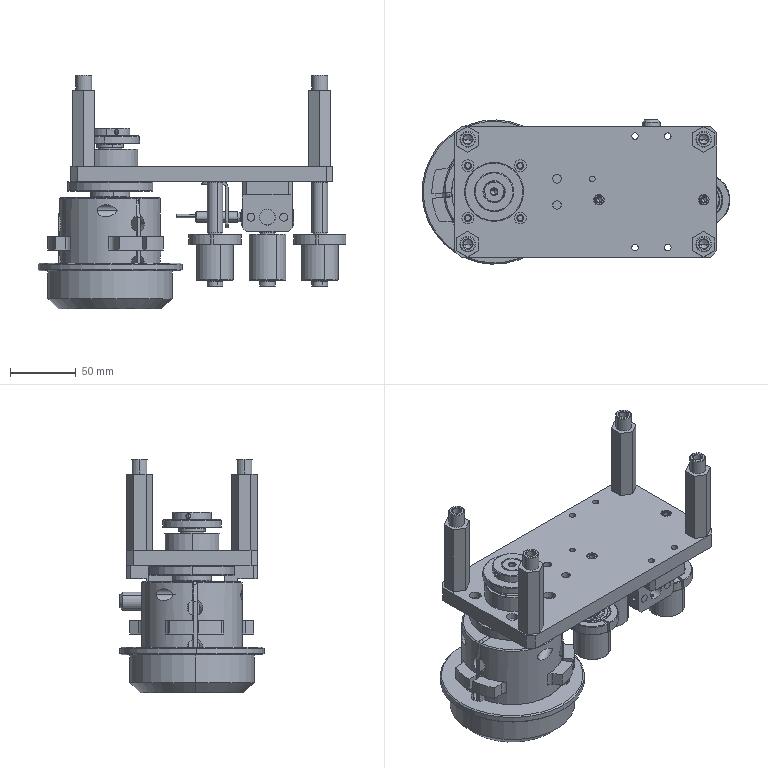Assembly | SolidWorks | mm | 39 component files | 95 solids | 1291 faces | box 235 x 110 x 178.5 mm | volume 896661 mm3 | cylinder 488 | plane 301 | cone 285 | spline 214 | torus 3 | commonest cylinder face diameters 12 x89 4.2 x28 9 x26 3.3 x26 24 x24 19.68 x24 16.32 x24 5 x22
Bill of materials:
61901Bearing | 6 | 45#Steel | Annular assembly of concentric outer and inner rings with flat faces, separated by an open annular gap holding six spherical elements spaced around it; looks like an open (unshielded) ball-bearing shape.
61904Bearing | 2 | 45#Steel | Same type of shape as the previous part: concentric inner and outer rings with six spheres in the annular gap between them, forming an open ball-bearing-like ring set.
YX-04-110GluePaperFeedingPressureRollerAxis | 2 | Hard Chrome Rod | Long stepped cylindrical shaft with a shorter, smaller-diameter end and an axial blind bore in the small end. The larger body has two narrow circumferential grooves: one around mid-length and one near the far end.
YX-04-111GluePaperRetainingRing | 2 | 45#Steel | Flat split ring with a rectangular cross-section, a single radial cut through the ring, and chamfered edges; looks like a split washer or split collar.
YX-04-112GluePaperFeedingBearingFixingSleeve | 3 | 45#Steel | Thin-walled cylindrical sleeve or bushing with an internal step near one end: a slightly larger counterbore at the top opening and a through bore.
YX-04-113GluePaperFeedingTensioningWheelFixingBlock | 2 | 45#Steel | Prismatic block with an L-shaped side profile. The top flange has two vertical through holes. The front face has one large central hole flanked by two medium holes. There are additional small holes, including one on the side leg, and chamfers on the lower corners.
YX-04-114GluePaperFeedingTensioningWheelAdjustingPost | 1 | 45#Steel | Stepped hollow cylindrical bushing or spacer: a larger-diameter body with a chamfer at one end and a smaller-diameter neck at the other. The axial bore opens at the small end.
YX-04-115GluePaperFeedingTensioningWheelGuideSleeve | 2 | Brass | Plain cylindrical tube or spacer with a concentric through bore and chamfered outer edges at both ends.
YX-04-116GluePaperFeedingTensioningWheelGuidePost | 2 | Hard Chrome Rod | Slender solid cylindrical rod or pin with plain flat ends and very small edge breaks.
YX-04-117GluePaperFeedingTensioningWheelFixingPlate | 1 | 45#Steel | Rectangular block with chamfered long edges, two large parallel through bores along one axis, and one smaller through hole on a perpendicular axis set midway between them.
YX-04-118GluePaperFeedingTensioningWheelAxis | 1 | 45#Steel | Stepped cylindrical shaft with a smaller-diameter end portion containing an axial bore, and a larger main body with narrow circumferential grooves near both ends.
PR8-2DN_1ProximitySwitch | 1 | 45#Steel | Solid stepped cylindrical rod: a thin small-diameter pin extending from a larger cylindrical body, which ends in a short, slightly reduced-diameter pilot step with a chamfer.
YX-04-102GluePaperFeedingColumn | 4 | Brass | Long hexagonal prism body with a shorter, smaller-diameter cylindrical boss coaxial at each end; a bore runs in from the top boss end, and the end view shows a recessed hole with a conical bottom.
YX-04-103GluePaperFeedingBottomPlate | 1 | 45#Steel | Flat rectangular plate with small chamfered corners, a large circular through-opening near one end, and many smaller through-holes of several sizes.
YX-04-104GluePaperFeedingBearingFixingSeat | 1 | 45#Steel | Flanged cylindrical sleeve: a thin round flange with four through-holes evenly spaced on a circle, and a taller hollow cylinder rising from it with an internal step in the bore.
YX-04-105GluePaperFeedingSensingBlock | 1 | 45#Steel | Stepped round hub: a wide thin disc with a smaller coaxial cylindrical boss on top, a central through-bore, and radial holes through the boss wall.
YX-04-106GluePaperFeedingRotatingAxis | 1 | 45#Steel | Stepped cylindrical shaft or pin with a thin integral collar near mid-length, a smaller-diameter pilot at the top end with a small axial hole, and a narrow groove or step near the upper shoulder.
YX-04-107GluePaperFeedingExpansionAxis | 1 | 45#Steel | Cylindrical body with a central axial bore, three outward-projecting lugs at mid-height, three radial slots on the top face, an axial slit through the side, a circumferential slot, and several radial and transverse holes.
YX-04-108GluePaperFeedingExpansionAxisCoverPlate | 1 | 45#Steel | Shallow round cup or cap with an outer lip flange at the top, a chamfered bottom edge, an internal cylindrical recess with two semicircular notches at its rim, and a small central hole in the floor.
YX-04-109GluePaperFeedingExpansionPlate | 3 | Delrin | Flat bar plate with two obround slots near the ends; one long edge is tapered toward each end and the corners on that side are rounded.
YX-04-119GlueFeedingProximitySwitchFixingPlate | 1 | SUS340 | L-shaped bracket bent from flat stock with a rounded inside bend; one leg has an elongated slot, the other a single round hole, and the free corners are rounded.
Mates:
1. concentric | YX-04-103GluePaperFeedingBottomPlate-1 face at (-123.397, -33.738, 194) dir (0, 0, -1) r 6 | YX-04-102GluePaperFeedingColumn-1 face at (-123.397, -33.738, 264) dir (0, 0, 1) r 6
2. concentric | YX-04-106GluePaperFeedingRotatingAxis-1 face at (-103.397, 6.262, 112) dir (0, 0, 1) r 10 | YX-04-107GluePaperFeedingExpansionAxis-1 face at (-103.397, 6.262, 182) dir (0, 0, 1) r 10
3. coincident | YX-04-106GluePaperFeedingRotatingAxis-1 face at (-103.397, 6.262, 112) dir (0, 0, -1) | YX-04-107GluePaperFeedingExpansionAxis-1 face at (-103.397, 6.262, 112) dir (0, 0, -1)
4. concentric | YX-04-106GluePaperFeedingRotatingAxis-1 face at (-103.397, 6.262, 112) dir (0, 0, -1) r 3.4 | YX-04-108GluePaperFeedingExpansionAxisCoverPlate-1 face at (-103.397, 6.262, 97) dir (0, 0, -1) r 4.5
5. width | YX-04-109GluePaperFeedingExpansionPlate-1 face at (-86.886, 36.162, 179) dir (0.8958, -0.4445, 0) | YX-04-109GluePaperFeedingExpansionPlate-1 face at (-89.573, 37.496, 179) dir (-0.8958, 0.4445, 0) | YX-04-107GluePaperFeedingExpansionAxis-1 face at (-75.16, 59.231, 112) dir (-0.8958, 0.4445, 0) | YX-04-107GluePaperFeedingExpansionAxis-1 face at (-96.075, 24.955, 112) dir (0.8958, -0.4445, 0)
6. width | YX-04-109GluePaperFeedingExpansionPlate-1 face at (-87.348, 35.23, 124.5) dir (0, 0, -1) | YX-04-109GluePaperFeedingExpansionPlate-1 face at (-88.682, 32.543, 119.5) dir (0, 0, 1) | YX-04-107GluePaperFeedingExpansionAxis-1 face at (-64.224, 20.314, 122) dir (0.8958, -0.4445, 0) r 2.75
7. coincident | YX-04-107GluePaperFeedingExpansionAxis-1 face at (-103.397, 6.262, 112) dir (0, 0, -1) | YX-04-109GluePaperFeedingExpansionPlate-1 face at (-86.886, 36.162, 112) dir (0, 0, -1)
8. coincident | YX-04-103GluePaperFeedingBottomPlate-1 face at (-33.397, 6.262, 206) dir (0, 0, 1) | YX-04-102GluePaperFeedingColumn-1 face at (-123.397, -33.738, 206) dir (0, 0, -1)
9. concentric | YX-04-106GluePaperFeedingRotatingAxis-1 face at (-103.397, 6.262, 235) dir (0, 0, -1) r 8 | YX-04-105GluePaperFeedingSensingBlock-1 face at (-103.397, 6.262, 235) dir (0, 0, 1) r 8
10. coincident | YX-04-103GluePaperFeedingBottomPlate-1 face at (-33.397, 6.262, 194) dir (0, 0, -1) | GluePaperFeedingPressureRollerAssembly-1/YX-04-110GluePaperFeedingPressureRollerAxis-1 face at (-18.121, 1.815, 194) dir (0, 0, 1)
11. concentric | YX-04-103GluePaperFeedingBottomPlate-1 face at (-23.397, 0.262, 194) dir (0, 0, -1) r 4 | GluePaperFeedingPressureRollerAssembly-1/YX-04-110GluePaperFeedingPressureRollerAxis-1 face at (-23.397, 0.262, 205.5) dir (0, 0, -1) r 6
12. coincident | YX-04-103GluePaperFeedingBottomPlate-1 face at (-33.397, 6.262, 194) dir (0, 0, -1) | GluePaperFeedingTensioningWheelAssembly-1/YX-04-113GluePaperFeedingTensioningWheelFixingBlock-2 face at (-2.397, 31.262, 194) dir (0, 0, 1)
13. concentric | YX-04-103GluePaperFeedingBottomPlate-1 face at (4.103, 48.762, 194) dir (0, 0, -1) r 2.5 | GluePaperFeedingTensioningWheelAssembly-1/YX-04-113GluePaperFeedingTensioningWheelFixingBlock-2 face at (4.103, 48.762, 194) dir (0, 0, 1) r 3.25
14. concentric | YX-04-103GluePaperFeedingBottomPlate-1 face at (29.103, 48.762, 194) dir (0, 0, -1) r 2.5 | GluePaperFeedingTensioningWheelAssembly-1/YX-04-113GluePaperFeedingTensioningWheelFixingBlock-2 face at (29.103, 48.762, 184) dir (0, 0, -1) r 3.25
15. coincident | YX-04-103GluePaperFeedingBottomPlate-1 face at (-33.397, 6.262, 194) dir (0, 0, -1) | YX-04-119GlueFeedingProximitySwitchFixingPlate-1 face at (-13.397, 14.462, 194) dir (0, 0, 1)
16. width | YX-04-119GlueFeedingProximitySwitchFixingPlate-1 face at (-25.797, 21.962, 159) dir (-1, 0, 0) | YX-04-119GlueFeedingProximitySwitchFixingPlate-1 face at (-30.997, 31.962, 159) dir (1, 0, 0) | YX-04-103GluePaperFeedingBottomPlate-1 face at (-28.397, 16.262, 194) dir (0, 0, -1) r 2.1
17. parallel | GluePaperFeedingTensioningWheelAssembly-1/YX-04-113GluePaperFeedingTensioningWheelFixingBlock-2 face at (-2.397, 31.262, 156) dir (-1, 0, 0) | YX-04-119GlueFeedingProximitySwitchFixingPlate-1 face at (-33.397, 26.962, 194) dir (-1, 0, 0)
18. distance | YX-04-103GluePaperFeedingBottomPlate-1 face at (-28.397, 16.262, 194) dir (0, 0, -1) r 2.1 | YX-04-119GlueFeedingProximitySwitchFixingPlate-1 face at (-28.397, 21.962, 159) dir (0, 0, 1) r 2.6
19. concentric | YX-04-119GlueFeedingProximitySwitchFixingPlate-1 face at (-13.397, 26.962, 167) dir (1, 0, 0) r 4.25 | PR8-2DN_1ProximitySwitch-1 face at (-5.897, 26.962, 167) dir (-1, 0, 0) r 4
20. distance | PR8-2DN_1ProximitySwitch-1 face at (-3.397, 26.962, 167) dir (1, 0, 0) | YX-04-119GlueFeedingProximitySwitchFixingPlate-1 face at (-13.397, 26.962, 194) dir (1, 0, 0)
21. coincident | GluePaperFeedingTensioningWheelAssembly-1/YX-04-112GluePaperFeedingBearingFixingSleeve-1 face at (26.976, 26.795, 125) dir (0, 0, -1) | 61901Bearing-2 face at (16.603, 20.762, 125) dir (0, 0, 1)
22. concentric | GluePaperFeedingTensioningWheelAssembly-1/YX-04-112GluePaperFeedingBearingFixingSleeve-1 face at (16.603, 20.762, 119) dir (0, 0, 1) r 12 | 61901Bearing-2 face at (16.603, 20.762, 118.7) dir (0, 0, 1) r 12
23. coincident | GluePaperFeedingTensioningWheelAssembly-1/YX-04-118GluePaperFeedingTensioningWheelAxis-1 face at (16.603, 26.762, 154) dir (0, 0, 1) | 61901Bearing-3 face at (16.603, 20.762, 154) dir (0, 0, 1)
24. concentric | GluePaperFeedingTensioningWheelAssembly-1/YX-04-118GluePaperFeedingTensioningWheelAxis-1 face at (16.603, 20.762, 174) dir (0, 0, -1) r 6 | 61901Bearing-3 face at (16.603, 20.762, 147.7) dir (0, 0, 1) r 6
25. coincident | YX-04-104GluePaperFeedingBearingFixingSeat-1 face at (-103.397, 22.262, 210) dir (0, 0, 1) | 61904Bearing-1 face at (-103.397, 6.262, 210) dir (0, 0, -1)
26. concentric | YX-04-104GluePaperFeedingBearingFixingSeat-1 face at (-103.397, 6.262, 219) dir (0, 0, -1) r 18.5 | 61904Bearing-1 face at (-103.397, 6.262, 219.45) dir (0, 0, -1) r 18.5
27. coincident | YX-04-104GluePaperFeedingBearingFixingSeat-1 face at (-103.397, 24.762, 196) dir (0, 0, -1) | 61904Bearing-2 face at (-103.397, 6.262, 196) dir (0, 0, 1)
28. concentric | YX-04-104GluePaperFeedingBearingFixingSeat-1 face at (-103.397, 6.262, 219) dir (0, 0, -1) r 18.5 | 61904Bearing-2 face at (-103.397, 6.262, 196.45) dir (0, 0, -1) r 18.5
29. coincident | YX-04-103GluePaperFeedingBottomPlate-1 face at (-33.397, 6.262, 194) dir (0, 0, -1) | YX-04-104GluePaperFeedingBearingFixingSeat-1 face at (-103.397, 38.762, 194) dir (0, 0, 1)
30. concentric | YX-04-103GluePaperFeedingBottomPlate-1 face at (-83.397, 26.262, 206) dir (0, 0, 1) r 2.75 | YX-04-104GluePaperFeedingBearingFixingSeat-1 face at (-83.397, 26.262, 194) dir (0, 0, 1) r 2.1
31. concentric | YX-04-103GluePaperFeedingBottomPlate-1 face at (-123.397, 26.262, 206) dir (0, 0, 1) r 2.75 | YX-04-104GluePaperFeedingBearingFixingSeat-1 face at (-123.397, 26.262, 194) dir (0, 0, 1) r 2.1
32. coincident | YX-04-106GluePaperFeedingRotatingAxis-1 face at (-118.176, 3.698, 187) dir (0, 0, 1) | 61904Bearing-2 face at (-103.397, 6.262, 187) dir (0, 0, -1)
33. width | YX-04-112GluePaperFeedingBearingFixingSleeve-1 face at (21.45, 22.403, 91.5) dir (1, 0, 0) | YX-04-112GluePaperFeedingBearingFixingSleeve-1 face at (-13.55, 24.003, 91.5) dir (-1, 0, 0) | YX-04-110GluePaperFeedingPressureRollerAxis-1 face at (21.45, 15.703, 91.5) dir (1, 0, 0) | YX-04-110GluePaperFeedingPressureRollerAxis-1 face at (-13.55, 16.203, 91.5) dir (-1, 0, 0)
34. concentric | YX-04-110GluePaperFeedingPressureRollerAxis-1 face at (-65.05, 10.203, 91.5) dir (1, 0, 0) r 6 | YX-04-112GluePaperFeedingBearingFixingSleeve-1 face at (-13.55, 10.203, 91.5) dir (1, 0, 0) r 14
35. coincident | YX-04-112GluePaperFeedingBearingFixingSleeve-1 face at (-13.55, 24.003, 91.5) dir (-1, 0, 0) | YX-04-111GluePaperRetainingRing-1 face at (-13.55, 10.203, 91.5) dir (-1, 0, 0)
36. concentric | YX-04-112GluePaperFeedingBearingFixingSleeve-1 face at (-13.55, 10.203, 91.5) dir (1, 0, 0) r 14 | YX-04-111GluePaperRetainingRing-1 face at (-13.55, 10.203, 91.5) dir (1, 0, 0) r 14
37. coincident | YX-04-112GluePaperFeedingBearingFixingSleeve-1 face at (15.45, 20.203, 91.5) dir (1, 0, 0) | 61901Bearing-1 face at (15.45, 10.203, 91.5) dir (-1, 0, 0)
38. concentric | YX-04-112GluePaperFeedingBearingFixingSleeve-1 face at (-13.55, 10.203, 91.5) dir (1, 0, 0) r 12 | 61901Bearing-1 face at (15.15, 10.203, 91.5) dir (1, 0, 0) r 12
39. coincident | YX-04-112GluePaperFeedingBearingFixingSleeve-1 face at (-7.55, 22.203, 91.5) dir (-1, 0, 0) | 61901Bearing-2 face at (-7.55, 10.203, 91.5) dir (1, 0, 0)
40. concentric | YX-04-112GluePaperFeedingBearingFixingSleeve-1 face at (-13.55, 10.203, 91.5) dir (1, 0, 0) r 12 | 61901Bearing-2 face at (-13.85, 10.203, 91.5) dir (1, 0, 0) r 12
41. concentric | YX-04-113GluePaperFeedingTensioningWheelFixingBlock-1 face at (-12.549, 8.675, 50.5) dir (1, 0, 0) r 3 | YX-04-116GluePaperFeedingTensioningWheelGuidePost-1 face at (-12.549, 8.675, 50.5) dir (-1, 0, 0) r 3
42. concentric | YX-04-116GluePaperFeedingTensioningWheelGuidePost-1 face at (-12.549, 8.675, 50.5) dir (-1, 0, 0) r 3 | YX-04-115GluePaperFeedingTensioningWheelGuideSleeve-1 face at (-67.549, 8.675, 50.5) dir (1, 0, 0) r 6
43. distance | YX-04-113GluePaperFeedingTensioningWheelFixingBlock-1 face at (-22.549, -18.325, 38) dir (-1, 0, 0) | YX-04-115GluePaperFeedingTensioningWheelGuideSleeve-1 face at (-48.549, 12.175, 50.5) dir (1, 0, 0)
44. coincident | YX-04-116GluePaperFeedingTensioningWheelGuidePost-1 face at (-82.549, 8.675, 50.5) dir (-1, 0, 0) | YX-04-113GluePaperFeedingTensioningWheelFixingBlock-2 face at (-82.549, 19.675, 57) dir (-1, 0, 0)
45. concentric | YX-04-116GluePaperFeedingTensioningWheelGuidePost-1 face at (-12.549, 8.675, 50.5) dir (-1, 0, 0) r 3 | YX-04-113GluePaperFeedingTensioningWheelFixingBlock-2 face at (-82.549, 8.675, 50.5) dir (-1, 0, 0) r 3
46. concentric | YX-04-116GluePaperFeedingTensioningWheelGuidePost-2 face at (-12.549, 8.675, 25.5) dir (-1, 0, 0) r 3 | YX-04-113GluePaperFeedingTensioningWheelFixingBlock-2 face at (-82.549, 8.675, 25.5) dir (-1, 0, 0) r 3
47. coincident | YX-04-113GluePaperFeedingTensioningWheelFixingBlock-1 face at (-12.549, 19.675, 19) dir (1, 0, 0) | YX-04-116GluePaperFeedingTensioningWheelGuidePost-1 face at (-12.549, 7.53, 53.273) dir (1, 0, 0)
48. concentric | YX-04-115GluePaperFeedingTensioningWheelGuideSleeve-1 face at (-67.549, 8.675, 50.5) dir (1, 0, 0) r 6 | YX-04-117GluePaperFeedingTensioningWheelFixingPlate-1 face at (-68.049, 8.675, 50.5) dir (-1, 0, 0) r 6
49. coincident | YX-04-117GluePaperFeedingTensioningWheelFixingPlate-1 face at (-58.049, 16.675, 38) dir (0, 1, 0) | YX-04-118GluePaperFeedingTensioningWheelAxis-1 face at (-67.549, 16.675, 38) dir (0, -1, 0)
50. concentric | YX-04-117GluePaperFeedingTensioningWheelFixingPlate-1 face at (-62.049, 0.6753, 38) dir (0, -1, 0) r 4 | YX-04-118GluePaperFeedingTensioningWheelAxis-1 face at (-62.049, 1.675, 38) dir (0, 1, 0) r 4
51. concentric | YX-04-118GluePaperFeedingTensioningWheelAxis-1 face at (-62.049, 1.675, 38) dir (0, 1, 0) r 6 | YX-04-112GluePaperFeedingBearingFixingSleeve-1 face at (-62.049, 56.675, 38) dir (0, -1, 0) r 10
52. concentric | YX-04-115GluePaperFeedingTensioningWheelGuideSleeve-2 face at (-67.549, 8.675, 25.5) dir (1, 0, 0) r 6 | YX-04-117GluePaperFeedingTensioningWheelFixingPlate-1 face at (-48.049, 8.675, 25.5) dir (1, 0, 0) r 6
53. width | YX-04-112GluePaperFeedingBearingFixingSleeve-1 face at (-68.987, 56.675, 49.929) dir (0, 1, 0) | YX-04-112GluePaperFeedingBearingFixingSleeve-1 face at (-68.183, 21.675, 48.546) dir (0, -1, 0) | YX-04-118GluePaperFeedingTensioningWheelAxis-1 face at (-67.549, 56.675, 38) dir (0, 1, 0) | YX-04-118GluePaperFeedingTensioningWheelAxis-1 face at (-68.049, 21.675, 38) dir (0, -1, 0)
54. coincident | YX-04-113GluePaperFeedingTensioningWheelFixingBlock-2 face at (-82.549, 19.675, 57) dir (-1, 0, 0) | YX-04-114GluePaperFeedingTensioningWheelAdjustingPost-1 face at (-82.549, 3.385, 42.272) dir (1, 0, 0)
55. concentric | YX-04-113GluePaperFeedingTensioningWheelFixingBlock-2 face at (-82.549, 8.675, 38) dir (-1, 0, 0) r 6 | YX-04-114GluePaperFeedingTensioningWheelAdjustingPost-1 face at (-72.549, 8.675, 38) dir (-1, 0, 0) r 7
56. width | YX-04-115GluePaperFeedingTensioningWheelGuideSleeve-2 face at (-67.549, 14.175, 25.5) dir (-1, 0, 0) | YX-04-115GluePaperFeedingTensioningWheelGuideSleeve-2 face at (-48.549, 12.175, 25.5) dir (1, 0, 0) | YX-04-117GluePaperFeedingTensioningWheelFixingPlate-1 face at (-48.049, 0.6753, 58) dir (1, 0, 0) | YX-04-117GluePaperFeedingTensioningWheelFixingPlate-1 face at (-68.049, 0.6753, 18) dir (-1, 0, 0)